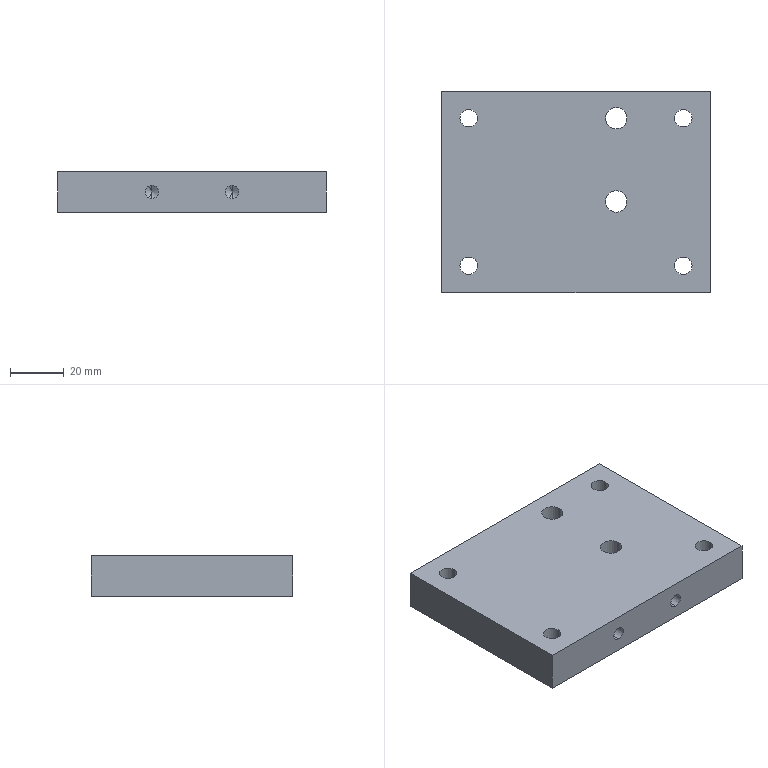Component | SolidWorks | JL001-05-05-003-1 | 1 solid | 26 faces | box 100 x 75 x 15 mm | volume 108392 mm3 | cylinder 16 | plane 6 | cone 4 | commonest cylinder face diameters 6.5 x8 5 x4 8 x4
build123d program:
from build123d import *

# Parameters (mm, degrees)
SKETCH1_W                  = 100
SKETCH1_H                  = 75
BOSS_EXTRUDE1_DEPTH        = 7.5
M8_TAPPED_HOLE1_D          = 8
F_6_5_6_5_DIAMETER_HOLE1_D = 6.5
M6_TAPPED_HOLE1_D          = 5
M6_TAPPED_HOLE1_DEPTH      = 15
M6_TAPPED_HOLE1_TIP        = 1.502


with BuildPart() as part:
    # Sketch1 → Boss-Extrude1 (new, symmetric)
    with BuildSketch(Plane.XY):
        Rectangle(SKETCH1_W, SKETCH1_H)
    extrude(amount=BOSS_EXTRUDE1_DEPTH, both=True)

    # M8 Tapped Hole1 (through all)
    with Locations(Plane.XY.offset(7.5)):
        with Locations((15, 27.5), (15, -3.5)):
            Hole(M8_TAPPED_HOLE1_D / 2)

    # 6.5 _6.5_ Diameter Hole1 (through all)
    with Locations(Plane.XY.offset(7.5)):
        with Locations((-40, 27.5), (-40, -27.5), (40, 27.5), (40, -27.5)):
            Hole(F_6_5_6_5_DIAMETER_HOLE1_D / 2)

    # M6 Tapped Hole1
    with Locations(Plane(origin=(0, -37.5, 0), x_dir=(-1, 0, 0), z_dir=(0, -1, 0))):
        with Locations((15, 0), (-15, 0)):
            Hole(M6_TAPPED_HOLE1_D / 2, depth=M6_TAPPED_HOLE1_DEPTH)
            with Locations((0, 0, -(M6_TAPPED_HOLE1_DEPTH + M6_TAPPED_HOLE1_TIP / 2))):  # 118° drill point
                Cone(0, M6_TAPPED_HOLE1_D / 2, M6_TAPPED_HOLE1_TIP, mode=Mode.SUBTRACT)


solid = part.part
STEP:
#1=CARTESIAN_POINT('',(-0.5906,-0.8858,0.09843));
#2=VERTEX_POINT('',#1);
#3=CARTESIAN_POINT('',(-0.5906,-0.8858,-0.09843));
#4=VERTEX_POINT('',#3);
#5=CARTESIAN_POINT('',(-0.5906,-0.8858,0.));
#6=DIRECTION('',(0.,-1.,0.));
#7=DIRECTION('',(0.,0.,-1.));
#8=AXIS2_PLACEMENT_3D('',#5,#6,#7);
#9=CIRCLE('',#8,0.09843);
#10=EDGE_CURVE('',#2,#4,#9,.T.);
#11=ORIENTED_EDGE('',*,*,#10,.F.);
#12=CARTESIAN_POINT('',(-0.5906,-1.476,0.09843));
#13=VERTEX_POINT('',#12);
#14=CARTESIAN_POINT('',(-0.5906,-1.476,0.09843));
#15=DIRECTION('',(0.,-1.,0.));
#16=VECTOR('',#15,39.37);
#17=LINE('',#14,#16);
#18=EDGE_CURVE('',#2,#13,#17,.T.);
#19=ORIENTED_EDGE('',*,*,#18,.T.);
#20=CARTESIAN_POINT('',(-0.5906,-1.476,-0.09843));
#21=VERTEX_POINT('',#20);
#22=CARTESIAN_POINT('',(-0.5906,-1.476,0.));
#23=DIRECTION('',(0.,-1.,0.));
#24=DIRECTION('',(0.,0.,-1.));
#25=AXIS2_PLACEMENT_3D('',#22,#23,#24);
#26=CIRCLE('',#25,0.09843);
#27=EDGE_CURVE('',#13,#21,#26,.T.);
#28=ORIENTED_EDGE('',*,*,#27,.T.);
#29=CARTESIAN_POINT('',(-0.5906,-1.476,-0.09843));
#30=DIRECTION('',(0.,-1.,0.));
#31=VECTOR('',#30,39.37);
#32=LINE('',#29,#31);
#33=EDGE_CURVE('',#4,#21,#32,.T.);
#34=ORIENTED_EDGE('',*,*,#33,.F.);
#35=EDGE_LOOP('',(#11,#19,#28,#34));
#36=FACE_OUTER_BOUND('',#35,.T.);
#37=CARTESIAN_POINT('',(-0.5906,-1.476,0.));
#38=DIRECTION('',(0.,-1.,0.));
#39=DIRECTION('',(0.,0.,-1.));
#40=AXIS2_PLACEMENT_3D('',#37,#38,#39);
#41=CYLINDRICAL_SURFACE('',#40,0.09843);
#42=ADVANCED_FACE('',(#36),#41,.F.);
#43=CARTESIAN_POINT('',(-0.5906,-0.8267,0.));
#44=VERTEX_POINT('',#43);
#45=CARTESIAN_POINT('',(-0.5906,-0.8858,-0.09843));
#46=DIRECTION('',(0.,-0.515,-0.8572));
#47=VECTOR('',#46,39.37);
#48=LINE('',#45,#47);
#49=EDGE_CURVE('',#44,#4,#48,.T.);
#50=ORIENTED_EDGE('',*,*,#49,.F.);
#51=CARTESIAN_POINT('',(-0.5906,-0.8858,0.09843));
#52=DIRECTION('',(0.,-0.515,0.8572));
#53=VECTOR('',#52,39.37);
#54=LINE('',#51,#53);
#55=EDGE_CURVE('',#44,#2,#54,.T.);
#56=ORIENTED_EDGE('',*,*,#55,.T.);
#57=ORIENTED_EDGE('',*,*,#10,.T.);
#58=EDGE_LOOP('',(#50,#56,#57));
#59=FACE_OUTER_BOUND('',#58,.T.);
#60=CARTESIAN_POINT('',(-0.5906,-0.8858,0.));
#61=DIRECTION('',(0.,-1.,0.));
#62=DIRECTION('',(0.,0.,-1.));
#63=AXIS2_PLACEMENT_3D('',#60,#61,#62);
#64=CONICAL_SURFACE('',#63,0.09843,1.03);
#65=ADVANCED_FACE('',(#59),#64,.F.);
#66=CARTESIAN_POINT('',(0.5906,-0.8858,0.09843));
#67=VERTEX_POINT('',#66);
#68=CARTESIAN_POINT('',(0.5906,-0.8858,-0.09843));
#69=VERTEX_POINT('',#68);
#70=CARTESIAN_POINT('',(0.5906,-0.8858,0.));
#71=DIRECTION('',(0.,-1.,0.));
#72=DIRECTION('',(0.,0.,-1.));
#73=AXIS2_PLACEMENT_3D('',#70,#71,#72);
#74=CIRCLE('',#73,0.09843);
#75=EDGE_CURVE('',#67,#69,#74,.T.);
#76=ORIENTED_EDGE('',*,*,#75,.F.);
#77=CARTESIAN_POINT('',(0.5906,-1.476,0.09843));
#78=VERTEX_POINT('',#77);
#79=CARTESIAN_POINT('',(0.5906,-1.476,0.09843));
#80=DIRECTION('',(0.,-1.,0.));
#81=VECTOR('',#80,39.37);
#82=LINE('',#79,#81);
#83=EDGE_CURVE('',#67,#78,#82,.T.);
#84=ORIENTED_EDGE('',*,*,#83,.T.);
#85=CARTESIAN_POINT('',(0.5906,-1.476,-0.09843));
#86=VERTEX_POINT('',#85);
#87=CARTESIAN_POINT('',(0.5906,-1.476,0.));
#88=DIRECTION('',(0.,-1.,0.));
#89=DIRECTION('',(0.,0.,-1.));
#90=AXIS2_PLACEMENT_3D('',#87,#88,#89);
#91=CIRCLE('',#90,0.09843);
#92=EDGE_CURVE('',#78,#86,#91,.T.);
#93=ORIENTED_EDGE('',*,*,#92,.T.);
#94=CARTESIAN_POINT('',(0.5906,-1.476,-0.09843));
#95=DIRECTION('',(0.,-1.,0.));
#96=VECTOR('',#95,39.37);
#97=LINE('',#94,#96);
#98=EDGE_CURVE('',#69,#86,#97,.T.);
#99=ORIENTED_EDGE('',*,*,#98,.F.);
#100=EDGE_LOOP('',(#76,#84,#93,#99));
#101=FACE_OUTER_BOUND('',#100,.T.);
#102=CARTESIAN_POINT('',(0.5906,-1.476,0.));
#103=DIRECTION('',(0.,-1.,0.));
#104=DIRECTION('',(0.,0.,-1.));
#105=AXIS2_PLACEMENT_3D('',#102,#103,#104);
#106=CYLINDRICAL_SURFACE('',#105,0.09843);
#107=ADVANCED_FACE('',(#101),#106,.F.);
#108=CARTESIAN_POINT('',(0.5906,-0.8267,0.));
#109=VERTEX_POINT('',#108);
#110=CARTESIAN_POINT('',(0.5906,-0.8858,-0.09843));
#111=DIRECTION('',(0.,-0.515,-0.8572));
#112=VECTOR('',#111,39.37);
#113=LINE('',#110,#112);
#114=EDGE_CURVE('',#109,#69,#113,.T.);
#115=ORIENTED_EDGE('',*,*,#114,.F.);
#116=CARTESIAN_POINT('',(0.5906,-0.8858,0.09843));
#117=DIRECTION('',(0.,-0.515,0.8572));
#118=VECTOR('',#117,39.37);
#119=LINE('',#116,#118);
#120=EDGE_CURVE('',#109,#67,#119,.T.);
#121=ORIENTED_EDGE('',*,*,#120,.T.);
#122=ORIENTED_EDGE('',*,*,#75,.T.);
#123=EDGE_LOOP('',(#115,#121,#122));
#124=FACE_OUTER_BOUND('',#123,.T.);
#125=CARTESIAN_POINT('',(0.5906,-0.8858,0.));
#126=DIRECTION('',(0.,-1.,0.));
#127=DIRECTION('',(0.,0.,-1.));
#128=AXIS2_PLACEMENT_3D('',#125,#126,#127);
#129=CONICAL_SURFACE('',#128,0.09843,1.03);
#130=ADVANCED_FACE('',(#124),#129,.F.);
#131=CARTESIAN_POINT('',(-1.703,1.083,-0.2953));
#132=VERTEX_POINT('',#131);
#133=CARTESIAN_POINT('',(-1.447,1.083,-0.2953));
#134=VERTEX_POINT('',#133);
#135=CARTESIAN_POINT('',(-1.575,1.083,-0.2953));
#136=DIRECTION('',(0.,0.,1.));
#137=DIRECTION('',(1.,0.,0.));
#138=AXIS2_PLACEMENT_3D('',#135,#136,#137);
#139=CIRCLE('',#138,0.128);
#140=EDGE_CURVE('',#132,#134,#139,.T.);
#141=ORIENTED_EDGE('',*,*,#140,.F.);
#142=CARTESIAN_POINT('',(-1.703,1.083,0.2953));
#143=VERTEX_POINT('',#142);
#144=CARTESIAN_POINT('',(-1.703,1.083,0.2953));
#145=DIRECTION('',(0.,0.,1.));
#146=VECTOR('',#145,39.37);
#147=LINE('',#144,#146);
#148=EDGE_CURVE('',#132,#143,#147,.T.);
#149=ORIENTED_EDGE('',*,*,#148,.T.);
#150=CARTESIAN_POINT('',(-1.447,1.083,0.2953));
#151=VERTEX_POINT('',#150);
#152=CARTESIAN_POINT('',(-1.575,1.083,0.2953));
#153=DIRECTION('',(0.,0.,1.));
#154=DIRECTION('',(1.,0.,0.));
#155=AXIS2_PLACEMENT_3D('',#152,#153,#154);
#156=CIRCLE('',#155,0.128);
#157=EDGE_CURVE('',#143,#151,#156,.T.);
#158=ORIENTED_EDGE('',*,*,#157,.T.);
#159=CARTESIAN_POINT('',(-1.447,1.083,0.2953));
#160=DIRECTION('',(0.,0.,1.));
#161=VECTOR('',#160,39.37);
#162=LINE('',#159,#161);
#163=EDGE_CURVE('',#134,#151,#162,.T.);
#164=ORIENTED_EDGE('',*,*,#163,.F.);
#165=EDGE_LOOP('',(#141,#149,#158,#164));
#166=FACE_OUTER_BOUND('',#165,.T.);
#167=CARTESIAN_POINT('',(-1.575,1.083,0.2953));
#168=DIRECTION('',(0.,0.,1.));
#169=DIRECTION('',(1.,0.,0.));
#170=AXIS2_PLACEMENT_3D('',#167,#168,#169);
#171=CYLINDRICAL_SURFACE('',#170,0.128);
#172=ADVANCED_FACE('',(#166),#171,.F.);
#173=CARTESIAN_POINT('',(-1.703,-1.083,-0.2953));
#174=VERTEX_POINT('',#173);
#175=CARTESIAN_POINT('',(-1.447,-1.083,-0.2953));
#176=VERTEX_POINT('',#175);
#177=CARTESIAN_POINT('',(-1.575,-1.083,-0.2953));
#178=DIRECTION('',(0.,0.,1.));
#179=DIRECTION('',(1.,0.,0.));
#180=AXIS2_PLACEMENT_3D('',#177,#178,#179);
#181=CIRCLE('',#180,0.128);
#182=EDGE_CURVE('',#174,#176,#181,.T.);
#183=ORIENTED_EDGE('',*,*,#182,.F.);
#184=CARTESIAN_POINT('',(-1.703,-1.083,0.2953));
#185=VERTEX_POINT('',#184);
#186=CARTESIAN_POINT('',(-1.703,-1.083,0.2953));
#187=DIRECTION('',(0.,0.,1.));
#188=VECTOR('',#187,39.37);
#189=LINE('',#186,#188);
#190=EDGE_CURVE('',#174,#185,#189,.T.);
#191=ORIENTED_EDGE('',*,*,#190,.T.);
#192=CARTESIAN_POINT('',(-1.447,-1.083,0.2953));
#193=VERTEX_POINT('',#192);
#194=CARTESIAN_POINT('',(-1.575,-1.083,0.2953));
#195=DIRECTION('',(0.,0.,1.));
#196=DIRECTION('',(1.,0.,0.));
#197=AXIS2_PLACEMENT_3D('',#194,#195,#196);
#198=CIRCLE('',#197,0.128);
#199=EDGE_CURVE('',#185,#193,#198,.T.);
#200=ORIENTED_EDGE('',*,*,#199,.T.);
#201=CARTESIAN_POINT('',(-1.447,-1.083,0.2953));
#202=DIRECTION('',(0.,0.,1.));
#203=VECTOR('',#202,39.37);
#204=LINE('',#201,#203);
#205=EDGE_CURVE('',#176,#193,#204,.T.);
#206=ORIENTED_EDGE('',*,*,#205,.F.);
#207=EDGE_LOOP('',(#183,#191,#200,#206));
#208=FACE_OUTER_BOUND('',#207,.T.);
#209=CARTESIAN_POINT('',(-1.575,-1.083,0.2953));
#210=DIRECTION('',(0.,0.,1.));
#211=DIRECTION('',(1.,0.,0.));
#212=AXIS2_PLACEMENT_3D('',#209,#210,#211);
#213=CYLINDRICAL_SURFACE('',#212,0.128);
#214=ADVANCED_FACE('',(#208),#213,.F.);
#215=CARTESIAN_POINT('',(1.447,1.083,-0.2953));
#216=VERTEX_POINT('',#215);
#217=CARTESIAN_POINT('',(1.703,1.083,-0.2953));
#218=VERTEX_POINT('',#217);
#219=CARTESIAN_POINT('',(1.575,1.083,-0.2953));
#220=DIRECTION('',(0.,0.,1.));
#221=DIRECTION('',(1.,0.,0.));
#222=AXIS2_PLACEMENT_3D('',#219,#220,#221);
#223=CIRCLE('',#222,0.128);
#224=EDGE_CURVE('',#216,#218,#223,.T.);
#225=ORIENTED_EDGE('',*,*,#224,.F.);
#226=CARTESIAN_POINT('',(1.447,1.083,0.2953));
#227=VERTEX_POINT('',#226);
#228=CARTESIAN_POINT('',(1.447,1.083,0.2953));
#229=DIRECTION('',(0.,0.,1.));
#230=VECTOR('',#229,39.37);
#231=LINE('',#228,#230);
#232=EDGE_CURVE('',#216,#227,#231,.T.);
#233=ORIENTED_EDGE('',*,*,#232,.T.);
#234=CARTESIAN_POINT('',(1.703,1.083,0.2953));
#235=VERTEX_POINT('',#234);
#236=CARTESIAN_POINT('',(1.575,1.083,0.2953));
#237=DIRECTION('',(0.,0.,1.));
#238=DIRECTION('',(1.,0.,0.));
#239=AXIS2_PLACEMENT_3D('',#236,#237,#238);
#240=CIRCLE('',#239,0.128);
#241=EDGE_CURVE('',#227,#235,#240,.T.);
#242=ORIENTED_EDGE('',*,*,#241,.T.);
#243=CARTESIAN_POINT('',(1.703,1.083,0.2953));
#244=DIRECTION('',(0.,0.,1.));
#245=VECTOR('',#244,39.37);
#246=LINE('',#243,#245);
#247=EDGE_CURVE('',#218,#235,#246,.T.);
#248=ORIENTED_EDGE('',*,*,#247,.F.);
#249=EDGE_LOOP('',(#225,#233,#242,#248));
#250=FACE_OUTER_BOUND('',#249,.T.);
#251=CARTESIAN_POINT('',(1.575,1.083,0.2953));
#252=DIRECTION('',(0.,0.,1.));
#253=DIRECTION('',(1.,0.,0.));
#254=AXIS2_PLACEMENT_3D('',#251,#252,#253);
#255=CYLINDRICAL_SURFACE('',#254,0.128);
#256=ADVANCED_FACE('',(#250),#255,.F.);
#257=CARTESIAN_POINT('',(1.447,-1.083,-0.2953));
#258=VERTEX_POINT('',#257);
#259=CARTESIAN_POINT('',(1.703,-1.083,-0.2953));
#260=VERTEX_POINT('',#259);
#261=CARTESIAN_POINT('',(1.575,-1.083,-0.2953));
#262=DIRECTION('',(0.,0.,1.));
#263=DIRECTION('',(1.,0.,0.));
#264=AXIS2_PLACEMENT_3D('',#261,#262,#263);
#265=CIRCLE('',#264,0.128);
#266=EDGE_CURVE('',#258,#260,#265,.T.);
#267=ORIENTED_EDGE('',*,*,#266,.F.);
#268=CARTESIAN_POINT('',(1.447,-1.083,0.2953));
#269=VERTEX_POINT('',#268);
#270=CARTESIAN_POINT('',(1.447,-1.083,0.2953));
#271=DIRECTION('',(0.,0.,1.));
#272=VECTOR('',#271,39.37);
#273=LINE('',#270,#272);
#274=EDGE_CURVE('',#258,#269,#273,.T.);
#275=ORIENTED_EDGE('',*,*,#274,.T.);
#276=CARTESIAN_POINT('',(1.703,-1.083,0.2953));
#277=VERTEX_POINT('',#276);
#278=CARTESIAN_POINT('',(1.575,-1.083,0.2953));
#279=DIRECTION('',(0.,0.,1.));
#280=DIRECTION('',(1.,0.,0.));
#281=AXIS2_PLACEMENT_3D('',#278,#279,#280);
#282=CIRCLE('',#281,0.128);
#283=EDGE_CURVE('',#269,#277,#282,.T.);
#284=ORIENTED_EDGE('',*,*,#283,.T.);
#285=CARTESIAN_POINT('',(1.703,-1.083,0.2953));
#286=DIRECTION('',(0.,0.,1.));
#287=VECTOR('',#286,39.37);
#288=LINE('',#285,#287);
#289=EDGE_CURVE('',#260,#277,#288,.T.);
#290=ORIENTED_EDGE('',*,*,#289,.F.);
#291=EDGE_LOOP('',(#267,#275,#284,#290));
#292=FACE_OUTER_BOUND('',#291,.T.);
#293=CARTESIAN_POINT('',(1.575,-1.083,0.2953));
#294=DIRECTION('',(0.,0.,1.));
#295=DIRECTION('',(1.,0.,0.));
#296=AXIS2_PLACEMENT_3D('',#293,#294,#295);
#297=CYLINDRICAL_SURFACE('',#296,0.128);
#298=ADVANCED_FACE('',(#292),#297,.F.);
#299=CARTESIAN_POINT('',(0.4331,1.083,-0.2953));
#300=VERTEX_POINT('',#299);
#301=CARTESIAN_POINT('',(0.748,1.083,-0.2953));
#302=VERTEX_POINT('',#301);
#303=CARTESIAN_POINT('',(0.5906,1.083,-0.2953));
#304=DIRECTION('',(0.,0.,1.));
#305=DIRECTION('',(1.,0.,0.));
#306=AXIS2_PLACEMENT_3D('',#303,#304,#305);
#307=CIRCLE('',#306,0.1575);
#308=EDGE_CURVE('',#300,#302,#307,.T.);
#309=ORIENTED_EDGE('',*,*,#308,.F.);
#310=CARTESIAN_POINT('',(0.4331,1.083,0.2953));
#311=VERTEX_POINT('',#310);
#312=CARTESIAN_POINT('',(0.4331,1.083,0.2953));
#313=DIRECTION('',(0.,0.,1.));
#314=VECTOR('',#313,39.37);
#315=LINE('',#312,#314);
#316=EDGE_CURVE('',#300,#311,#315,.T.);
#317=ORIENTED_EDGE('',*,*,#316,.T.);
#318=CARTESIAN_POINT('',(0.748,1.083,0.2953));
#319=VERTEX_POINT('',#318);
#320=CARTESIAN_POINT('',(0.5906,1.083,0.2953));
#321=DIRECTION('',(0.,0.,1.));
#322=DIRECTION('',(1.,0.,0.));
#323=AXIS2_PLACEMENT_3D('',#320,#321,#322);
#324=CIRCLE('',#323,0.1575);
#325=EDGE_CURVE('',#311,#319,#324,.T.);
#326=ORIENTED_EDGE('',*,*,#325,.T.);
#327=CARTESIAN_POINT('',(0.748,1.083,0.2953));
#328=DIRECTION('',(0.,0.,1.));
#329=VECTOR('',#328,39.37);
#330=LINE('',#327,#329);
#331=EDGE_CURVE('',#302,#319,#330,.T.);
#332=ORIENTED_EDGE('',*,*,#331,.F.);
#333=EDGE_LOOP('',(#309,#317,#326,#332));
#334=FACE_OUTER_BOUND('',#333,.T.);
#335=CARTESIAN_POINT('',(0.5906,1.083,0.2953));
#336=DIRECTION('',(0.,0.,1.));
#337=DIRECTION('',(1.,0.,0.));
#338=AXIS2_PLACEMENT_3D('',#335,#336,#337);
#339=CYLINDRICAL_SURFACE('',#338,0.1575);
#340=ADVANCED_FACE('',(#334),#339,.F.);
#341=CARTESIAN_POINT('',(0.4331,-0.1378,-0.2953));
#342=VERTEX_POINT('',#341);
#343=CARTESIAN_POINT('',(0.748,-0.1378,-0.2953));
#344=VERTEX_POINT('',#343);
#345=CARTESIAN_POINT('',(0.5906,-0.1378,-0.2953));
#346=DIRECTION('',(0.,0.,1.));
#347=DIRECTION('',(1.,0.,0.));
#348=AXIS2_PLACEMENT_3D('',#345,#346,#347);
#349=CIRCLE('',#348,0.1575);
#350=EDGE_CURVE('',#342,#344,#349,.T.);
#351=ORIENTED_EDGE('',*,*,#350,.F.);
#352=CARTESIAN_POINT('',(0.4331,-0.1378,0.2953));
#353=VERTEX_POINT('',#352);
#354=CARTESIAN_POINT('',(0.4331,-0.1378,0.2953));
#355=DIRECTION('',(0.,0.,1.));
#356=VECTOR('',#355,39.37);
#357=LINE('',#354,#356);
#358=EDGE_CURVE('',#342,#353,#357,.T.);
#359=ORIENTED_EDGE('',*,*,#358,.T.);
#360=CARTESIAN_POINT('',(0.748,-0.1378,0.2953));
#361=VERTEX_POINT('',#360);
#362=CARTESIAN_POINT('',(0.5906,-0.1378,0.2953));
#363=DIRECTION('',(0.,0.,1.));
#364=DIRECTION('',(1.,0.,0.));
#365=AXIS2_PLACEMENT_3D('',#362,#363,#364);
#366=CIRCLE('',#365,0.1575);
#367=EDGE_CURVE('',#353,#361,#366,.T.);
#368=ORIENTED_EDGE('',*,*,#367,.T.);
#369=CARTESIAN_POINT('',(0.748,-0.1378,0.2953));
#370=DIRECTION('',(0.,0.,1.));
#371=VECTOR('',#370,39.37);
#372=LINE('',#369,#371);
#373=EDGE_CURVE('',#344,#361,#372,.T.);
#374=ORIENTED_EDGE('',*,*,#373,.F.);
#375=EDGE_LOOP('',(#351,#359,#368,#374));
#376=FACE_OUTER_BOUND('',#375,.T.);
#377=CARTESIAN_POINT('',(0.5906,-0.1378,0.2953));
#378=DIRECTION('',(0.,0.,1.));
#379=DIRECTION('',(1.,0.,0.));
#380=AXIS2_PLACEMENT_3D('',#377,#378,#379);
#381=CYLINDRICAL_SURFACE('',#380,0.1575);
#382=ADVANCED_FACE('',(#376),#381,.F.);
#383=CARTESIAN_POINT('',(1.969,-1.476,-0.2953));
#384=VERTEX_POINT('',#383);
#385=CARTESIAN_POINT('',(1.969,1.476,-0.2953));
#386=VERTEX_POINT('',#385);
#387=CARTESIAN_POINT('',(1.969,1.476,-0.2953));
#388=DIRECTION('',(0.,1.,0.));
#389=VECTOR('',#388,39.37);
#390=LINE('',#387,#389);
#391=EDGE_CURVE('',#384,#386,#390,.T.);
#392=ORIENTED_EDGE('',*,*,#391,.T.);
#393=CARTESIAN_POINT('',(1.969,1.476,0.2953));
#394=VERTEX_POINT('',#393);
#395=CARTESIAN_POINT('',(1.969,1.476,0.2953));
#396=DIRECTION('',(0.,0.,-1.));
#397=VECTOR('',#396,39.37);
#398=LINE('',#395,#397);
#399=EDGE_CURVE('',#394,#386,#398,.T.);
#400=ORIENTED_EDGE('',*,*,#399,.F.);
#401=CARTESIAN_POINT('',(1.969,-1.476,0.2953));
#402=VERTEX_POINT('',#401);
#403=CARTESIAN_POINT('',(1.969,1.476,0.2953));
#404=DIRECTION('',(0.,1.,0.));
#405=VECTOR('',#404,39.37);
#406=LINE('',#403,#405);
#407=EDGE_CURVE('',#402,#394,#406,.T.);
#408=ORIENTED_EDGE('',*,*,#407,.F.);
#409=CARTESIAN_POINT('',(1.969,-1.476,0.2953));
#410=DIRECTION('',(0.,0.,-1.));
#411=VECTOR('',#410,39.37);
#412=LINE('',#409,#411);
#413=EDGE_CURVE('',#402,#384,#412,.T.);
#414=ORIENTED_EDGE('',*,*,#413,.T.);
#415=EDGE_LOOP('',(#392,#400,#408,#414));
#416=FACE_OUTER_BOUND('',#415,.T.);
#417=CARTESIAN_POINT('',(1.969,1.476,0.2953));
#418=DIRECTION('',(-1.,0.,0.));
#419=DIRECTION('',(0.,0.,1.));
#420=AXIS2_PLACEMENT_3D('',#417,#418,#419);
#421=PLANE('',#420);
#422=ADVANCED_FACE('',(#416),#421,.F.);
#423=CARTESIAN_POINT('',(-1.969,1.476,-0.2953));
#424=VERTEX_POINT('',#423);
#425=CARTESIAN_POINT('',(-1.969,1.476,-0.2953));
#426=DIRECTION('',(-1.,0.,0.));
#427=VECTOR('',#426,39.37);
#428=LINE('',#425,#427);
#429=EDGE_CURVE('',#386,#424,#428,.T.);
#430=ORIENTED_EDGE('',*,*,#429,.T.);
#431=CARTESIAN_POINT('',(-1.969,1.476,0.2953));
#432=VERTEX_POINT('',#431);
#433=CARTESIAN_POINT('',(-1.969,1.476,0.2953));
#434=DIRECTION('',(0.,0.,-1.));
#435=VECTOR('',#434,39.37);
#436=LINE('',#433,#435);
#437=EDGE_CURVE('',#432,#424,#436,.T.);
#438=ORIENTED_EDGE('',*,*,#437,.F.);
#439=CARTESIAN_POINT('',(-1.969,1.476,0.2953));
#440=DIRECTION('',(-1.,0.,0.));
#441=VECTOR('',#440,39.37);
#442=LINE('',#439,#441);
#443=EDGE_CURVE('',#394,#432,#442,.T.);
#444=ORIENTED_EDGE('',*,*,#443,.F.);
#445=ORIENTED_EDGE('',*,*,#399,.T.);
#446=EDGE_LOOP('',(#430,#438,#444,#445));
#447=FACE_OUTER_BOUND('',#446,.T.);
#448=CARTESIAN_POINT('',(-1.969,1.476,0.2953));
#449=DIRECTION('',(0.,-1.,0.));
#450=DIRECTION('',(0.,0.,-1.));
#451=AXIS2_PLACEMENT_3D('',#448,#449,#450);
#452=PLANE('',#451);
#453=ADVANCED_FACE('',(#447),#452,.F.);
#454=CARTESIAN_POINT('',(-1.969,-1.476,-0.2953));
#455=VERTEX_POINT('',#454);
#456=CARTESIAN_POINT('',(-1.969,1.476,-0.2953));
#457=DIRECTION('',(0.,-1.,0.));
#458=VECTOR('',#457,39.37);
#459=LINE('',#456,#458);
#460=EDGE_CURVE('',#424,#455,#459,.T.);
#461=ORIENTED_EDGE('',*,*,#460,.T.);
#462=CARTESIAN_POINT('',(-1.969,-1.476,0.2953));
#463=VERTEX_POINT('',#462);
#464=CARTESIAN_POINT('',(-1.969,-1.476,0.2953));
#465=DIRECTION('',(0.,0.,-1.));
#466=VECTOR('',#465,39.37);
#467=LINE('',#464,#466);
#468=EDGE_CURVE('',#463,#455,#467,.T.);
#469=ORIENTED_EDGE('',*,*,#468,.F.);
#470=CARTESIAN_POINT('',(-1.969,1.476,0.2953));
#471=DIRECTION('',(0.,-1.,0.));
#472=VECTOR('',#471,39.37);
#473=LINE('',#470,#472);
#474=EDGE_CURVE('',#432,#463,#473,.T.);
#475=ORIENTED_EDGE('',*,*,#474,.F.);
#476=ORIENTED_EDGE('',*,*,#437,.T.);
#477=EDGE_LOOP('',(#461,#469,#475,#476));
#478=FACE_OUTER_BOUND('',#477,.T.);
#479=CARTESIAN_POINT('',(-1.969,1.476,0.2953));
#480=DIRECTION('',(1.,0.,0.));
#481=DIRECTION('',(-0.,1.,0.));
#482=AXIS2_PLACEMENT_3D('',#479,#480,#481);
#483=PLANE('',#482);
#484=ADVANCED_FACE('',(#478),#483,.F.);
#485=CARTESIAN_POINT('',(-0.5906,-1.476,0.));
#486=DIRECTION('',(0.,-1.,0.));
#487=DIRECTION('',(0.,0.,-1.));
#488=AXIS2_PLACEMENT_3D('',#485,#486,#487);
#489=CIRCLE('',#488,0.09843);
#490=EDGE_CURVE('',#21,#13,#489,.T.);
#491=ORIENTED_EDGE('',*,*,#490,.F.);
#492=ORIENTED_EDGE('',*,*,#27,.F.);
#493=EDGE_LOOP('',(#491,#492));
#494=FACE_BOUND('',#493,.T.);
#495=CARTESIAN_POINT('',(0.5906,-1.476,0.));
#496=DIRECTION('',(0.,-1.,0.));
#497=DIRECTION('',(0.,0.,-1.));
#498=AXIS2_PLACEMENT_3D('',#495,#496,#497);
#499=CIRCLE('',#498,0.09843);
#500=EDGE_CURVE('',#86,#78,#499,.T.);
#501=ORIENTED_EDGE('',*,*,#500,.F.);
#502=ORIENTED_EDGE('',*,*,#92,.F.);
#503=EDGE_LOOP('',(#501,#502));
#504=FACE_BOUND('',#503,.T.);
#505=CARTESIAN_POINT('',(-1.969,-1.476,-0.2953));
#506=DIRECTION('',(1.,0.,0.));
#507=VECTOR('',#506,39.37);
#508=LINE('',#505,#507);
#509=EDGE_CURVE('',#455,#384,#508,.T.);
#510=ORIENTED_EDGE('',*,*,#509,.T.);
#511=ORIENTED_EDGE('',*,*,#413,.F.);
#512=CARTESIAN_POINT('',(-1.969,-1.476,0.2953));
#513=DIRECTION('',(1.,0.,0.));
#514=VECTOR('',#513,39.37);
#515=LINE('',#512,#514);
#516=EDGE_CURVE('',#463,#402,#515,.T.);
#517=ORIENTED_EDGE('',*,*,#516,.F.);
#518=ORIENTED_EDGE('',*,*,#468,.T.);
#519=EDGE_LOOP('',(#510,#511,#517,#518));
#520=FACE_OUTER_BOUND('',#519,.T.);
#521=CARTESIAN_POINT('',(-1.969,-1.476,0.2953));
#522=DIRECTION('',(0.,1.,0.));
#523=DIRECTION('',(0.,0.,1.));
#524=AXIS2_PLACEMENT_3D('',#521,#522,#523);
#525=PLANE('',#524);
#526=ADVANCED_FACE('',(#494,#504,#520),#525,.F.);
#527=CARTESIAN_POINT('',(-1.575,1.083,0.2953));
#528=DIRECTION('',(0.,0.,1.));
#529=DIRECTION('',(1.,0.,0.));
#530=AXIS2_PLACEMENT_3D('',#527,#528,#529);
#531=CIRCLE('',#530,0.128);
#532=EDGE_CURVE('',#151,#143,#531,.T.);
#533=ORIENTED_EDGE('',*,*,#532,.F.);
#534=ORIENTED_EDGE('',*,*,#157,.F.);
#535=EDGE_LOOP('',(#533,#534));
#536=FACE_BOUND('',#535,.T.);
#537=CARTESIAN_POINT('',(-1.575,-1.083,0.2953));
#538=DIRECTION('',(0.,0.,1.));
#539=DIRECTION('',(1.,0.,0.));
#540=AXIS2_PLACEMENT_3D('',#537,#538,#539);
#541=CIRCLE('',#540,0.128);
#542=EDGE_CURVE('',#193,#185,#541,.T.);
#543=ORIENTED_EDGE('',*,*,#542,.F.);
#544=ORIENTED_EDGE('',*,*,#199,.F.);
#545=EDGE_LOOP('',(#543,#544));
#546=FACE_BOUND('',#545,.T.);
#547=CARTESIAN_POINT('',(1.575,1.083,0.2953));
#548=DIRECTION('',(0.,0.,1.));
#549=DIRECTION('',(1.,0.,0.));
#550=AXIS2_PLACEMENT_3D('',#547,#548,#549);
#551=CIRCLE('',#550,0.128);
#552=EDGE_CURVE('',#235,#227,#551,.T.);
#553=ORIENTED_EDGE('',*,*,#552,.F.);
#554=ORIENTED_EDGE('',*,*,#241,.F.);
#555=EDGE_LOOP('',(#553,#554));
#556=FACE_BOUND('',#555,.T.);
#557=CARTESIAN_POINT('',(1.575,-1.083,0.2953));
#558=DIRECTION('',(0.,0.,1.));
#559=DIRECTION('',(1.,0.,0.));
#560=AXIS2_PLACEMENT_3D('',#557,#558,#559);
#561=CIRCLE('',#560,0.128);
#562=EDGE_CURVE('',#277,#269,#561,.T.);
#563=ORIENTED_EDGE('',*,*,#562,.F.);
#564=ORIENTED_EDGE('',*,*,#283,.F.);
#565=EDGE_LOOP('',(#563,#564));
#566=FACE_BOUND('',#565,.T.);
#567=CARTESIAN_POINT('',(0.5906,1.083,0.2953));
#568=DIRECTION('',(0.,0.,1.));
#569=DIRECTION('',(1.,0.,0.));
#570=AXIS2_PLACEMENT_3D('',#567,#568,#569);
#571=CIRCLE('',#570,0.1575);
#572=EDGE_CURVE('',#319,#311,#571,.T.);
#573=ORIENTED_EDGE('',*,*,#572,.F.);
#574=ORIENTED_EDGE('',*,*,#325,.F.);
#575=EDGE_LOOP('',(#573,#574));
#576=FACE_BOUND('',#575,.T.);
#577=CARTESIAN_POINT('',(0.5906,-0.1378,0.2953));
#578=DIRECTION('',(0.,0.,1.));
#579=DIRECTION('',(1.,0.,0.));
#580=AXIS2_PLACEMENT_3D('',#577,#578,#579);
#581=CIRCLE('',#580,0.1575);
#582=EDGE_CURVE('',#361,#353,#581,.T.);
#583=ORIENTED_EDGE('',*,*,#582,.F.);
#584=ORIENTED_EDGE('',*,*,#367,.F.);
#585=EDGE_LOOP('',(#583,#584));
#586=FACE_BOUND('',#585,.T.);
#587=ORIENTED_EDGE('',*,*,#407,.T.);
#588=ORIENTED_EDGE('',*,*,#443,.T.);
#589=ORIENTED_EDGE('',*,*,#474,.T.);
#590=ORIENTED_EDGE('',*,*,#516,.T.);
#591=EDGE_LOOP('',(#587,#588,#589,#590));
#592=FACE_OUTER_BOUND('',#591,.T.);
#593=CARTESIAN_POINT('',(0.,0.,0.2953));
#594=DIRECTION('',(0.,0.,1.));
#595=DIRECTION('',(1.,0.,0.));
#596=AXIS2_PLACEMENT_3D('',#593,#594,#595);
#597=PLANE('',#596);
#598=ADVANCED_FACE('',(#536,#546,#556,#566,#576,#586,#592),#597,.T.);
#599=CARTESIAN_POINT('',(-1.575,1.083,-0.2953));
#600=DIRECTION('',(0.,0.,1.));
#601=DIRECTION('',(1.,0.,0.));
#602=AXIS2_PLACEMENT_3D('',#599,#600,#601);
#603=CIRCLE('',#602,0.128);
#604=EDGE_CURVE('',#134,#132,#603,.T.);
#605=ORIENTED_EDGE('',*,*,#604,.T.);
#606=ORIENTED_EDGE('',*,*,#140,.T.);
#607=EDGE_LOOP('',(#605,#606));
#608=FACE_BOUND('',#607,.T.);
#609=CARTESIAN_POINT('',(-1.575,-1.083,-0.2953));
#610=DIRECTION('',(0.,0.,1.));
#611=DIRECTION('',(1.,0.,0.));
#612=AXIS2_PLACEMENT_3D('',#609,#610,#611);
#613=CIRCLE('',#612,0.128);
#614=EDGE_CURVE('',#176,#174,#613,.T.);
#615=ORIENTED_EDGE('',*,*,#614,.T.);
#616=ORIENTED_EDGE('',*,*,#182,.T.);
#617=EDGE_LOOP('',(#615,#616));
#618=FACE_BOUND('',#617,.T.);
#619=CARTESIAN_POINT('',(1.575,1.083,-0.2953));
#620=DIRECTION('',(0.,0.,1.));
#621=DIRECTION('',(1.,0.,0.));
#622=AXIS2_PLACEMENT_3D('',#619,#620,#621);
#623=CIRCLE('',#622,0.128);
#624=EDGE_CURVE('',#218,#216,#623,.T.);
#625=ORIENTED_EDGE('',*,*,#624,.T.);
#626=ORIENTED_EDGE('',*,*,#224,.T.);
#627=EDGE_LOOP('',(#625,#626));
#628=FACE_BOUND('',#627,.T.);
#629=CARTESIAN_POINT('',(1.575,-1.083,-0.2953));
#630=DIRECTION('',(0.,0.,1.));
#631=DIRECTION('',(1.,0.,0.));
#632=AXIS2_PLACEMENT_3D('',#629,#630,#631);
#633=CIRCLE('',#632,0.128);
#634=EDGE_CURVE('',#260,#258,#633,.T.);
#635=ORIENTED_EDGE('',*,*,#634,.T.);
#636=ORIENTED_EDGE('',*,*,#266,.T.);
#637=EDGE_LOOP('',(#635,#636));
#638=FACE_BOUND('',#637,.T.);
#639=CARTESIAN_POINT('',(0.5906,1.083,-0.2953));
#640=DIRECTION('',(0.,0.,1.));
#641=DIRECTION('',(1.,0.,0.));
#642=AXIS2_PLACEMENT_3D('',#639,#640,#641);
#643=CIRCLE('',#642,0.1575);
#644=EDGE_CURVE('',#302,#300,#643,.T.);
#645=ORIENTED_EDGE('',*,*,#644,.T.);
#646=ORIENTED_EDGE('',*,*,#308,.T.);
#647=EDGE_LOOP('',(#645,#646));
#648=FACE_BOUND('',#647,.T.);
#649=CARTESIAN_POINT('',(0.5906,-0.1378,-0.2953));
#650=DIRECTION('',(0.,0.,1.));
#651=DIRECTION('',(1.,0.,0.));
#652=AXIS2_PLACEMENT_3D('',#649,#650,#651);
#653=CIRCLE('',#652,0.1575);
#654=EDGE_CURVE('',#344,#342,#653,.T.);
#655=ORIENTED_EDGE('',*,*,#654,.T.);
#656=ORIENTED_EDGE('',*,*,#350,.T.);
#657=EDGE_LOOP('',(#655,#656));
#658=FACE_BOUND('',#657,.T.);
#659=ORIENTED_EDGE('',*,*,#391,.F.);
#660=ORIENTED_EDGE('',*,*,#509,.F.);
#661=ORIENTED_EDGE('',*,*,#460,.F.);
#662=ORIENTED_EDGE('',*,*,#429,.F.);
#663=EDGE_LOOP('',(#659,#660,#661,#662));
#664=FACE_OUTER_BOUND('',#663,.T.);
#665=CARTESIAN_POINT('',(0.,0.,-0.2953));
#666=DIRECTION('',(0.,0.,1.));
#667=DIRECTION('',(1.,0.,0.));
#668=AXIS2_PLACEMENT_3D('',#665,#666,#667);
#669=PLANE('',#668);
#670=ADVANCED_FACE('',(#608,#618,#628,#638,#648,#658,#664),#669,.F.);
#671=ORIENTED_EDGE('',*,*,#358,.F.);
#672=ORIENTED_EDGE('',*,*,#654,.F.);
#673=ORIENTED_EDGE('',*,*,#373,.T.);
#674=ORIENTED_EDGE('',*,*,#582,.T.);
#675=EDGE_LOOP('',(#671,#672,#673,#674));
#676=FACE_OUTER_BOUND('',#675,.T.);
#677=CARTESIAN_POINT('',(0.5906,-0.1378,0.2953));
#678=DIRECTION('',(0.,0.,1.));
#679=DIRECTION('',(1.,0.,0.));
#680=AXIS2_PLACEMENT_3D('',#677,#678,#679);
#681=CYLINDRICAL_SURFACE('',#680,0.1575);
#682=ADVANCED_FACE('',(#676),#681,.F.);
#683=ORIENTED_EDGE('',*,*,#316,.F.);
#684=ORIENTED_EDGE('',*,*,#644,.F.);
#685=ORIENTED_EDGE('',*,*,#331,.T.);
#686=ORIENTED_EDGE('',*,*,#572,.T.);
#687=EDGE_LOOP('',(#683,#684,#685,#686));
#688=FACE_OUTER_BOUND('',#687,.T.);
#689=CARTESIAN_POINT('',(0.5906,1.083,0.2953));
#690=DIRECTION('',(0.,0.,1.));
#691=DIRECTION('',(1.,0.,0.));
#692=AXIS2_PLACEMENT_3D('',#689,#690,#691);
#693=CYLINDRICAL_SURFACE('',#692,0.1575);
#694=ADVANCED_FACE('',(#688),#693,.F.);
#695=ORIENTED_EDGE('',*,*,#274,.F.);
#696=ORIENTED_EDGE('',*,*,#634,.F.);
#697=ORIENTED_EDGE('',*,*,#289,.T.);
#698=ORIENTED_EDGE('',*,*,#562,.T.);
#699=EDGE_LOOP('',(#695,#696,#697,#698));
#700=FACE_OUTER_BOUND('',#699,.T.);
#701=CARTESIAN_POINT('',(1.575,-1.083,0.2953));
#702=DIRECTION('',(0.,0.,1.));
#703=DIRECTION('',(1.,0.,0.));
#704=AXIS2_PLACEMENT_3D('',#701,#702,#703);
#705=CYLINDRICAL_SURFACE('',#704,0.128);
#706=ADVANCED_FACE('',(#700),#705,.F.);
#707=ORIENTED_EDGE('',*,*,#232,.F.);
#708=ORIENTED_EDGE('',*,*,#624,.F.);
#709=ORIENTED_EDGE('',*,*,#247,.T.);
#710=ORIENTED_EDGE('',*,*,#552,.T.);
#711=EDGE_LOOP('',(#707,#708,#709,#710));
#712=FACE_OUTER_BOUND('',#711,.T.);
#713=CARTESIAN_POINT('',(1.575,1.083,0.2953));
#714=DIRECTION('',(0.,0.,1.));
#715=DIRECTION('',(1.,0.,0.));
#716=AXIS2_PLACEMENT_3D('',#713,#714,#715);
#717=CYLINDRICAL_SURFACE('',#716,0.128);
#718=ADVANCED_FACE('',(#712),#717,.F.);
#719=ORIENTED_EDGE('',*,*,#190,.F.);
#720=ORIENTED_EDGE('',*,*,#614,.F.);
#721=ORIENTED_EDGE('',*,*,#205,.T.);
#722=ORIENTED_EDGE('',*,*,#542,.T.);
#723=EDGE_LOOP('',(#719,#720,#721,#722));
#724=FACE_OUTER_BOUND('',#723,.T.);
#725=CARTESIAN_POINT('',(-1.575,-1.083,0.2953));
#726=DIRECTION('',(0.,0.,1.));
#727=DIRECTION('',(1.,0.,0.));
#728=AXIS2_PLACEMENT_3D('',#725,#726,#727);
#729=CYLINDRICAL_SURFACE('',#728,0.128);
#730=ADVANCED_FACE('',(#724),#729,.F.);
#731=ORIENTED_EDGE('',*,*,#148,.F.);
#732=ORIENTED_EDGE('',*,*,#604,.F.);
#733=ORIENTED_EDGE('',*,*,#163,.T.);
#734=ORIENTED_EDGE('',*,*,#532,.T.);
#735=EDGE_LOOP('',(#731,#732,#733,#734));
#736=FACE_OUTER_BOUND('',#735,.T.);
#737=CARTESIAN_POINT('',(-1.575,1.083,0.2953));
#738=DIRECTION('',(0.,0.,1.));
#739=DIRECTION('',(1.,0.,0.));
#740=AXIS2_PLACEMENT_3D('',#737,#738,#739);
#741=CYLINDRICAL_SURFACE('',#740,0.128);
#742=ADVANCED_FACE('',(#736),#741,.F.);
#743=ORIENTED_EDGE('',*,*,#120,.F.);
#744=ORIENTED_EDGE('',*,*,#114,.T.);
#745=CARTESIAN_POINT('',(0.5906,-0.8858,0.));
#746=DIRECTION('',(0.,-1.,0.));
#747=DIRECTION('',(0.,0.,-1.));
#748=AXIS2_PLACEMENT_3D('',#745,#746,#747);
#749=CIRCLE('',#748,0.09843);
#750=EDGE_CURVE('',#69,#67,#749,.T.);
#751=ORIENTED_EDGE('',*,*,#750,.T.);
#752=EDGE_LOOP('',(#743,#744,#751));
#753=FACE_OUTER_BOUND('',#752,.T.);
#754=CARTESIAN_POINT('',(0.5906,-0.8858,0.));
#755=DIRECTION('',(0.,-1.,0.));
#756=DIRECTION('',(0.,0.,-1.));
#757=AXIS2_PLACEMENT_3D('',#754,#755,#756);
#758=CONICAL_SURFACE('',#757,0.09843,1.03);
#759=ADVANCED_FACE('',(#753),#758,.F.);
#760=ORIENTED_EDGE('',*,*,#83,.F.);
#761=ORIENTED_EDGE('',*,*,#750,.F.);
#762=ORIENTED_EDGE('',*,*,#98,.T.);
#763=ORIENTED_EDGE('',*,*,#500,.T.);
#764=EDGE_LOOP('',(#760,#761,#762,#763));
#765=FACE_OUTER_BOUND('',#764,.T.);
#766=CARTESIAN_POINT('',(0.5906,-1.476,0.));
#767=DIRECTION('',(0.,-1.,0.));
#768=DIRECTION('',(0.,0.,-1.));
#769=AXIS2_PLACEMENT_3D('',#766,#767,#768);
#770=CYLINDRICAL_SURFACE('',#769,0.09843);
#771=ADVANCED_FACE('',(#765),#770,.F.);
#772=ORIENTED_EDGE('',*,*,#55,.F.);
#773=ORIENTED_EDGE('',*,*,#49,.T.);
#774=CARTESIAN_POINT('',(-0.5906,-0.8858,0.));
#775=DIRECTION('',(0.,-1.,0.));
#776=DIRECTION('',(0.,0.,-1.));
#777=AXIS2_PLACEMENT_3D('',#774,#775,#776);
#778=CIRCLE('',#777,0.09843);
#779=EDGE_CURVE('',#4,#2,#778,.T.);
#780=ORIENTED_EDGE('',*,*,#779,.T.);
#781=EDGE_LOOP('',(#772,#773,#780));
#782=FACE_OUTER_BOUND('',#781,.T.);
#783=CARTESIAN_POINT('',(-0.5906,-0.8858,0.));
#784=DIRECTION('',(0.,-1.,0.));
#785=DIRECTION('',(0.,0.,-1.));
#786=AXIS2_PLACEMENT_3D('',#783,#784,#785);
#787=CONICAL_SURFACE('',#786,0.09843,1.03);
#788=ADVANCED_FACE('',(#782),#787,.F.);
#789=ORIENTED_EDGE('',*,*,#18,.F.);
#790=ORIENTED_EDGE('',*,*,#779,.F.);
#791=ORIENTED_EDGE('',*,*,#33,.T.);
#792=ORIENTED_EDGE('',*,*,#490,.T.);
#793=EDGE_LOOP('',(#789,#790,#791,#792));
#794=FACE_OUTER_BOUND('',#793,.T.);
#795=CARTESIAN_POINT('',(-0.5906,-1.476,0.));
#796=DIRECTION('',(0.,-1.,0.));
#797=DIRECTION('',(0.,0.,-1.));
#798=AXIS2_PLACEMENT_3D('',#795,#796,#797);
#799=CYLINDRICAL_SURFACE('',#798,0.09843);
#800=ADVANCED_FACE('',(#794),#799,.F.);
#801=CLOSED_SHELL('',(#42,#65,#107,#130,#172,#214,#256,#298,#340,#382,#422,#453,#484,#526,#598,#670,#682,#694,#706,#718,#730,#742,#759,#771,#788,#800));
#802=MANIFOLD_SOLID_BREP('',#801);
#803=CARTESIAN_POINT('',(0.,0.,0.));
#804=DIRECTION('',(0.,0.,1.));
#805=DIRECTION('',(1.,0.,0.));
#806=AXIS2_PLACEMENT_3D('',#803,#804,#805);
#807=(LENGTH_UNIT()NAMED_UNIT(*)SI_UNIT($,.METRE.));
#808=LENGTH_MEASURE_WITH_UNIT(LENGTH_MEASURE(0.0254),#807);
#809=DIMENSIONAL_EXPONENTS(1.,0.,0.,0.,0.,0.,0.);
#810=(CONVERSION_BASED_UNIT('',#808)LENGTH_UNIT()NAMED_UNIT(#809));
#811=UNCERTAINTY_MEASURE_WITH_UNIT(LENGTH_MEASURE(0.00001),#810,'','');
#812=(NAMED_UNIT(*)PLANE_ANGLE_UNIT()SI_UNIT($,.RADIAN.));
#813=(NAMED_UNIT(*)SI_UNIT($,.STERADIAN.)SOLID_ANGLE_UNIT());
#814=(GEOMETRIC_REPRESENTATION_CONTEXT(3)GLOBAL_UNCERTAINTY_ASSIGNED_CONTEXT((#811))GLOBAL_UNIT_ASSIGNED_CONTEXT((#810,#812,#813))REPRESENTATION_CONTEXT('',''));
#815=ADVANCED_BREP_SHAPE_REPRESENTATION('',(#802,#806),#814);
#816=COLOUR_RGB('',0.7922,0.8196,0.9333);
#817=FILL_AREA_STYLE_COLOUR('',#816);
#818=FILL_AREA_STYLE('',(#817));
#819=SURFACE_STYLE_FILL_AREA(#818);
#820=SURFACE_SIDE_STYLE('',(#819));
#821=SURFACE_STYLE_USAGE(.BOTH.,#820);
#822=PRESENTATION_STYLE_ASSIGNMENT((#821));
#823=STYLED_ITEM('',(#822),#802);
#824=PRESENTATION_LAYER_ASSIGNMENT('','',(#823));
#825=(LENGTH_UNIT()NAMED_UNIT(*)SI_UNIT($,.METRE.));
#826=LENGTH_MEASURE_WITH_UNIT(LENGTH_MEASURE(0.0254),#825);
#827=DIMENSIONAL_EXPONENTS(1.,0.,0.,0.,0.,0.,0.);
#828=(CONVERSION_BASED_UNIT('',#826)LENGTH_UNIT()NAMED_UNIT(#827));
#829=UNCERTAINTY_MEASURE_WITH_UNIT(LENGTH_MEASURE(0.00001),#828,'','');
#830=(NAMED_UNIT(*)PLANE_ANGLE_UNIT()SI_UNIT($,.RADIAN.));
#831=(NAMED_UNIT(*)SI_UNIT($,.STERADIAN.)SOLID_ANGLE_UNIT());
#832=(GEOMETRIC_REPRESENTATION_CONTEXT(3)GLOBAL_UNCERTAINTY_ASSIGNED_CONTEXT((#829))GLOBAL_UNIT_ASSIGNED_CONTEXT((#828,#830,#831))REPRESENTATION_CONTEXT('',''));
#833=MECHANICAL_DESIGN_GEOMETRIC_PRESENTATION_REPRESENTATION('',(#823),#832);